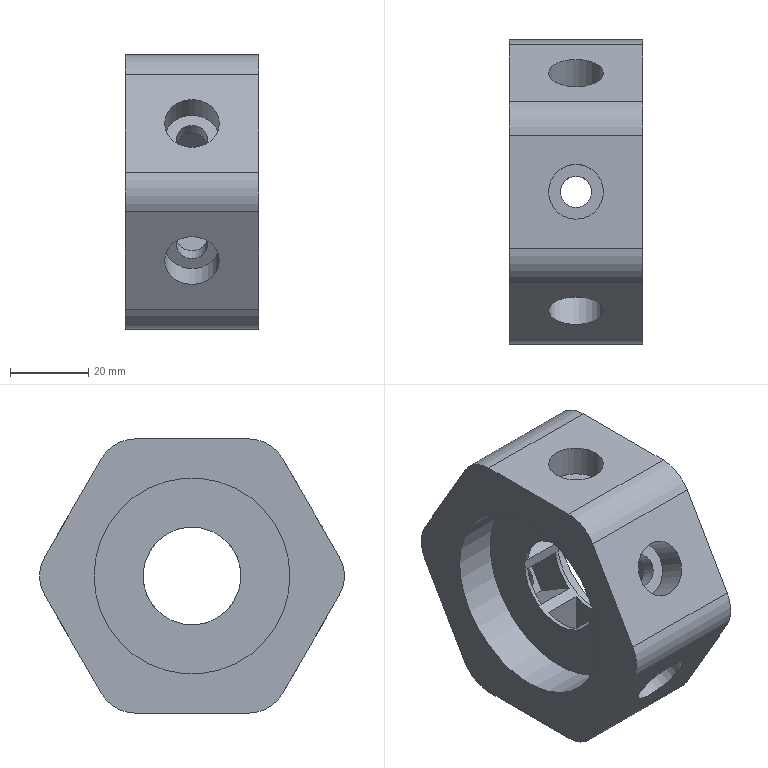Component | NX | SIX_SIDE_BODY | 1 solid | 67 faces | volume 78995 mm3 | plane 46 | cylinder 21 | commonest cylinder face diameters 20 x6 14 x6 8 x6 50 x2 25 x1